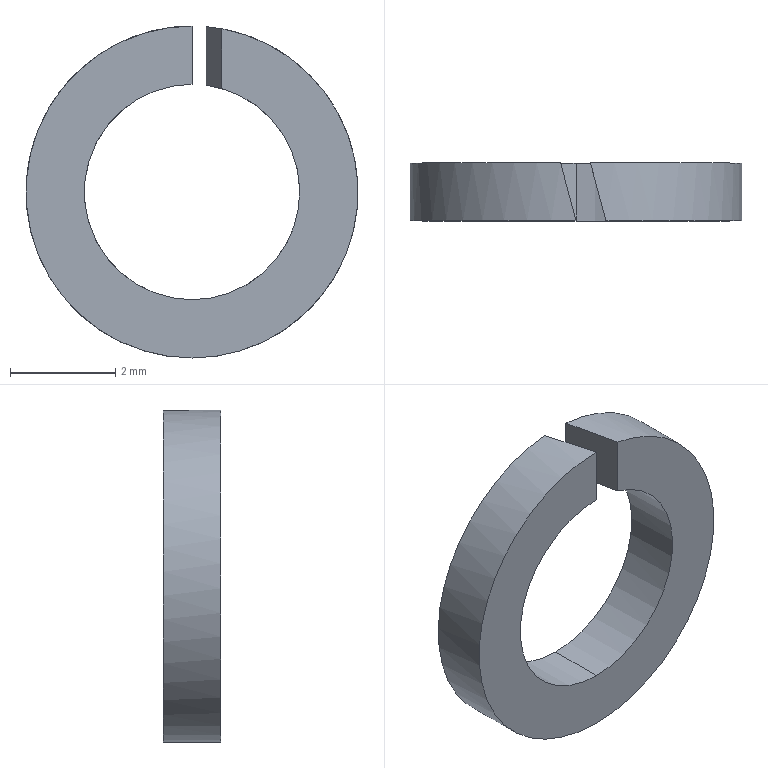Component | SolidWorks | GB 93-87-4-10 | 1 solid | 8 faces | box 6.32 x 1.1 x 6.32 mm | volume 19 mm3 | cylinder 4 | plane 4 | commonest cylinder face diameters 4.1 x2 6.32 x2
build123d program:
from build123d import *

# Parameters (mm, degrees)
SKETCH1_R               = 3.16
SKETCH1_R_2             = 2.05
BOSS_EXTRUDE1_DEPTH     = 1.1
CUT_EXTRUDE1_REACH      = 6.602
CUT_EXTRUDE1_END_RADIUS = 3.16


with BuildPart() as part:
    # Sketch1 → Boss-Extrude1 (new body)
    with BuildSketch(Plane(origin=(0, 0, 0), x_dir=(1, 0, 0), z_dir=(0, 1, 0))):
        with Locations(Location((0, 0, 0), (0, 0, 270))):
            Circle(SKETCH1_R)
        with Locations(Location((0, 0, 0), (0, 0, 270))):
            Circle(SKETCH1_R_2, mode=Mode.SUBTRACT)
    extrude(amount=BOSS_EXTRUDE1_DEPTH)

    # Cut-Extrude1: up to this cylinder (the profile starts inside it)
    cut_extrude1_end = Plane(origin=(0, 0.55, 0), z_dir=(0, -1, 0)) * Cylinder(CUT_EXTRUDE1_END_RADIUS, 20.524, mode=Mode.PRIVATE)
    # Sketch2 → Cut-Extrude1 (cut, up to the surface)
    with BuildSketch(Plane.XY, mode=Mode.PRIVATE) as cut_extrude1_sk1:
        Polygon((0, 0), (-0.2947, 1.1), (0.2747, 1.1), (0.5694, 0), align=None)
    cut_extrude1_tool1 = extrude(cut_extrude1_sk1.sketch, amount=CUT_EXTRUDE1_REACH, mode=Mode.PRIVATE) & cut_extrude1_end
    add(cut_extrude1_tool1.solids().sort_by_distance((0.1373, 0.55, 0))[0], mode=Mode.SUBTRACT)


solid = part.part

# Placed as in the assembly
solid = solid.moved(Location((-51.534, 76.366, -146.507), (0, 0, 0)))
STEP:
#1=COLOUR_RGB('',0.7922,0.8196,0.9333);
#2=FILL_AREA_STYLE_COLOUR('',#1);
#3=FILL_AREA_STYLE('',(#2));
#4=SURFACE_STYLE_FILL_AREA(#3);
#5=SURFACE_SIDE_STYLE('',(#4));
#6=SURFACE_STYLE_USAGE(.BOTH.,#5);
#7=PRESENTATION_STYLE_ASSIGNMENT((#6));
#8=CARTESIAN_POINT('',(-2.018,3.05,-5.688));
#9=VERTEX_POINT('',#8);
#10=CARTESIAN_POINT('',(-2.029,3.05,-5.849));
#11=VERTEX_POINT('',#10);
#12=CARTESIAN_POINT('',(-2.029,3.05,-5.768));
#13=DIRECTION('',(0.,1.,0.));
#14=DIRECTION('',(0.,0.,1.));
#15=AXIS2_PLACEMENT_3D('',#12,#13,#14);
#16=CIRCLE('',#15,0.08071);
#17=EDGE_CURVE('',#9,#11,#16,.T.);
#18=ORIENTED_EDGE('',*,*,#17,.T.);
#19=CARTESIAN_POINT('',(-2.029,3.007,-5.849));
#20=VERTEX_POINT('',#19);
#21=CARTESIAN_POINT('',(-2.029,3.05,-5.849));
#22=DIRECTION('',(0.,-1.,0.));
#23=VECTOR('',#22,39.37);
#24=LINE('',#21,#23);
#25=EDGE_CURVE('',#11,#20,#24,.T.);
#26=ORIENTED_EDGE('',*,*,#25,.T.);
#27=CARTESIAN_POINT('',(-2.006,3.007,-5.69));
#28=VERTEX_POINT('',#27);
#29=CARTESIAN_POINT('',(-2.029,3.007,-5.768));
#30=DIRECTION('',(0.,1.,0.));
#31=DIRECTION('',(0.,0.,1.));
#32=AXIS2_PLACEMENT_3D('',#29,#30,#31);
#33=CIRCLE('',#32,0.08071);
#34=EDGE_CURVE('',#28,#20,#33,.T.);
#35=ORIENTED_EDGE('',*,*,#34,.F.);
#36=CARTESIAN_POINT('',(-2.018,3.05,-5.688));
#37=CARTESIAN_POINT('',(-2.014,3.035,-5.689));
#38=CARTESIAN_POINT('',(-2.01,3.021,-5.689));
#39=CARTESIAN_POINT('',(-2.006,3.007,-5.69));
#40=(BOUNDED_CURVE()B_SPLINE_CURVE(3,(#36,#37,#38,#39),.UNSPECIFIED.,.F.,.F.)B_SPLINE_CURVE_WITH_KNOTS((4,4),(4.847,4.994),.UNSPECIFIED.)CURVE()GEOMETRIC_REPRESENTATION_ITEM()RATIONAL_B_SPLINE_CURVE((1.,0.9982,0.9982,1.))REPRESENTATION_ITEM(''));
#41=EDGE_CURVE('',#9,#28,#40,.T.);
#42=ORIENTED_EDGE('',*,*,#41,.F.);
#43=EDGE_LOOP('',(#18,#26,#35,#42));
#44=FACE_OUTER_BOUND('',#43,.T.);
#45=CARTESIAN_POINT('',(-2.029,3.05,-5.768));
#46=DIRECTION('',(0.,-1.,0.));
#47=DIRECTION('',(0.,0.,-1.));
#48=AXIS2_PLACEMENT_3D('',#45,#46,#47);
#49=CYLINDRICAL_SURFACE('',#48,0.08071);
#50=ADVANCED_FACE('',(#44),#49,.F.);
#51=CARTESIAN_POINT('',(-2.029,3.05,-5.892));
#52=VERTEX_POINT('',#51);
#53=CARTESIAN_POINT('',(-2.041,3.05,-5.644));
#54=VERTEX_POINT('',#53);
#55=CARTESIAN_POINT('',(-2.029,3.05,-5.768));
#56=DIRECTION('',(0.,1.,0.));
#57=DIRECTION('',(0.,0.,1.));
#58=AXIS2_PLACEMENT_3D('',#55,#56,#57);
#59=CIRCLE('',#58,0.1244);
#60=EDGE_CURVE('',#52,#54,#59,.T.);
#61=ORIENTED_EDGE('',*,*,#60,.F.);
#62=CARTESIAN_POINT('',(-2.029,3.007,-5.892));
#63=VERTEX_POINT('',#62);
#64=CARTESIAN_POINT('',(-2.029,3.05,-5.892));
#65=DIRECTION('',(0.,-1.,0.));
#66=VECTOR('',#65,39.37);
#67=LINE('',#64,#66);
#68=EDGE_CURVE('',#52,#63,#67,.T.);
#69=ORIENTED_EDGE('',*,*,#68,.T.);
#70=CARTESIAN_POINT('',(-2.029,3.007,-5.644));
#71=VERTEX_POINT('',#70);
#72=CARTESIAN_POINT('',(-2.029,3.007,-5.768));
#73=DIRECTION('',(0.,1.,0.));
#74=DIRECTION('',(0.,0.,1.));
#75=AXIS2_PLACEMENT_3D('',#72,#73,#74);
#76=CIRCLE('',#75,0.1244);
#77=EDGE_CURVE('',#63,#71,#76,.T.);
#78=ORIENTED_EDGE('',*,*,#77,.T.);
#79=CARTESIAN_POINT('',(-2.029,3.007,-5.644));
#80=CARTESIAN_POINT('',(-2.033,3.021,-5.644));
#81=CARTESIAN_POINT('',(-2.037,3.035,-5.644));
#82=CARTESIAN_POINT('',(-2.041,3.05,-5.644));
#83=(BOUNDED_CURVE()B_SPLINE_CURVE(3,(#79,#80,#81,#82),.UNSPECIFIED.,.F.,.F.)B_SPLINE_CURVE_WITH_KNOTS((4,4),(1.571,1.664),.UNSPECIFIED.)CURVE()GEOMETRIC_REPRESENTATION_ITEM()RATIONAL_B_SPLINE_CURVE((1.,0.9993,0.9993,1.))REPRESENTATION_ITEM(''));
#84=EDGE_CURVE('',#71,#54,#83,.T.);
#85=ORIENTED_EDGE('',*,*,#84,.T.);
#86=EDGE_LOOP('',(#61,#69,#78,#85));
#87=FACE_OUTER_BOUND('',#86,.T.);
#88=CARTESIAN_POINT('',(-2.029,3.05,-5.768));
#89=DIRECTION('',(0.,-1.,0.));
#90=DIRECTION('',(0.,0.,-1.));
#91=AXIS2_PLACEMENT_3D('',#88,#89,#90);
#92=CYLINDRICAL_SURFACE('',#91,0.1244);
#93=ADVANCED_FACE('',(#87),#92,.T.);
#94=ORIENTED_EDGE('',*,*,#17,.F.);
#95=CARTESIAN_POINT('',(-2.018,3.05,-5.644));
#96=VERTEX_POINT('',#95);
#97=CARTESIAN_POINT('',(-2.018,3.05,-5.644));
#98=DIRECTION('',(0.,0.,-1.));
#99=VECTOR('',#98,39.37);
#100=LINE('',#97,#99);
#101=EDGE_CURVE('',#96,#9,#100,.T.);
#102=ORIENTED_EDGE('',*,*,#101,.F.);
#103=CARTESIAN_POINT('',(-2.029,3.05,-5.768));
#104=DIRECTION('',(0.,1.,0.));
#105=DIRECTION('',(0.,0.,1.));
#106=AXIS2_PLACEMENT_3D('',#103,#104,#105);
#107=CIRCLE('',#106,0.1244);
#108=EDGE_CURVE('',#96,#52,#107,.T.);
#109=ORIENTED_EDGE('',*,*,#108,.T.);
#110=ORIENTED_EDGE('',*,*,#60,.T.);
#111=CARTESIAN_POINT('',(-2.041,3.05,-5.688));
#112=VERTEX_POINT('',#111);
#113=CARTESIAN_POINT('',(-2.041,3.05,-5.644));
#114=DIRECTION('',(0.,0.,-1.));
#115=VECTOR('',#114,39.37);
#116=LINE('',#113,#115);
#117=EDGE_CURVE('',#54,#112,#116,.T.);
#118=ORIENTED_EDGE('',*,*,#117,.T.);
#119=CARTESIAN_POINT('',(-2.029,3.05,-5.768));
#120=DIRECTION('',(0.,1.,0.));
#121=DIRECTION('',(0.,0.,1.));
#122=AXIS2_PLACEMENT_3D('',#119,#120,#121);
#123=CIRCLE('',#122,0.08071);
#124=EDGE_CURVE('',#11,#112,#123,.T.);
#125=ORIENTED_EDGE('',*,*,#124,.F.);
#126=EDGE_LOOP('',(#94,#102,#109,#110,#118,#125));
#127=FACE_OUTER_BOUND('',#126,.T.);
#128=CARTESIAN_POINT('',(-2.029,3.05,-5.768));
#129=DIRECTION('',(0.,1.,0.));
#130=DIRECTION('',(0.,0.,1.));
#131=AXIS2_PLACEMENT_3D('',#128,#129,#130);
#132=PLANE('',#131);
#133=ADVANCED_FACE('',(#127),#132,.T.);
#134=CARTESIAN_POINT('',(-2.006,3.007,-5.646));
#135=VERTEX_POINT('',#134);
#136=CARTESIAN_POINT('',(-2.006,3.007,-5.644));
#137=DIRECTION('',(0.,0.,-1.));
#138=VECTOR('',#137,39.37);
#139=LINE('',#136,#138);
#140=EDGE_CURVE('',#135,#28,#139,.T.);
#141=ORIENTED_EDGE('',*,*,#140,.T.);
#142=ORIENTED_EDGE('',*,*,#34,.T.);
#143=CARTESIAN_POINT('',(-2.029,3.007,-5.687));
#144=VERTEX_POINT('',#143);
#145=CARTESIAN_POINT('',(-2.029,3.007,-5.768));
#146=DIRECTION('',(0.,1.,0.));
#147=DIRECTION('',(0.,0.,1.));
#148=AXIS2_PLACEMENT_3D('',#145,#146,#147);
#149=CIRCLE('',#148,0.08071);
#150=EDGE_CURVE('',#20,#144,#149,.T.);
#151=ORIENTED_EDGE('',*,*,#150,.T.);
#152=CARTESIAN_POINT('',(-2.029,3.007,-5.644));
#153=DIRECTION('',(0.,0.,-1.));
#154=VECTOR('',#153,39.37);
#155=LINE('',#152,#154);
#156=EDGE_CURVE('',#71,#144,#155,.T.);
#157=ORIENTED_EDGE('',*,*,#156,.F.);
#158=ORIENTED_EDGE('',*,*,#77,.F.);
#159=CARTESIAN_POINT('',(-2.029,3.007,-5.768));
#160=DIRECTION('',(0.,1.,0.));
#161=DIRECTION('',(0.,0.,1.));
#162=AXIS2_PLACEMENT_3D('',#159,#160,#161);
#163=CIRCLE('',#162,0.1244);
#164=EDGE_CURVE('',#135,#63,#163,.T.);
#165=ORIENTED_EDGE('',*,*,#164,.F.);
#166=EDGE_LOOP('',(#141,#142,#151,#157,#158,#165));
#167=FACE_OUTER_BOUND('',#166,.T.);
#168=CARTESIAN_POINT('',(-2.029,3.007,-5.768));
#169=DIRECTION('',(0.,1.,0.));
#170=DIRECTION('',(0.,0.,1.));
#171=AXIS2_PLACEMENT_3D('',#168,#169,#170);
#172=PLANE('',#171);
#173=ADVANCED_FACE('',(#167),#172,.F.);
#174=ORIENTED_EDGE('',*,*,#68,.F.);
#175=ORIENTED_EDGE('',*,*,#108,.F.);
#176=CARTESIAN_POINT('',(-2.018,3.05,-5.644));
#177=CARTESIAN_POINT('',(-2.014,3.035,-5.644));
#178=CARTESIAN_POINT('',(-2.01,3.021,-5.645));
#179=CARTESIAN_POINT('',(-2.006,3.007,-5.646));
#180=(BOUNDED_CURVE()B_SPLINE_CURVE(3,(#176,#177,#178,#179),.UNSPECIFIED.,.F.,.F.)B_SPLINE_CURVE_WITH_KNOTS((4,4),(4.799,4.894),.UNSPECIFIED.)CURVE()GEOMETRIC_REPRESENTATION_ITEM()RATIONAL_B_SPLINE_CURVE((1.,0.9993,0.9993,1.))REPRESENTATION_ITEM(''));
#181=EDGE_CURVE('',#96,#135,#180,.T.);
#182=ORIENTED_EDGE('',*,*,#181,.T.);
#183=ORIENTED_EDGE('',*,*,#164,.T.);
#184=EDGE_LOOP('',(#174,#175,#182,#183));
#185=FACE_OUTER_BOUND('',#184,.T.);
#186=CARTESIAN_POINT('',(-2.029,3.05,-5.768));
#187=DIRECTION('',(0.,-1.,0.));
#188=DIRECTION('',(0.,0.,-1.));
#189=AXIS2_PLACEMENT_3D('',#186,#187,#188);
#190=CYLINDRICAL_SURFACE('',#189,0.1244);
#191=ADVANCED_FACE('',(#185),#190,.T.);
#192=ORIENTED_EDGE('',*,*,#25,.F.);
#193=ORIENTED_EDGE('',*,*,#124,.T.);
#194=CARTESIAN_POINT('',(-2.029,3.007,-5.687));
#195=CARTESIAN_POINT('',(-2.033,3.021,-5.687));
#196=CARTESIAN_POINT('',(-2.037,3.035,-5.688));
#197=CARTESIAN_POINT('',(-2.041,3.05,-5.688));
#198=(BOUNDED_CURVE()B_SPLINE_CURVE(3,(#194,#195,#196,#197),.UNSPECIFIED.,.F.,.F.)B_SPLINE_CURVE_WITH_KNOTS((4,4),(1.571,1.715),.UNSPECIFIED.)CURVE()GEOMETRIC_REPRESENTATION_ITEM()RATIONAL_B_SPLINE_CURVE((1.,0.9983,0.9983,1.))REPRESENTATION_ITEM(''));
#199=EDGE_CURVE('',#144,#112,#198,.T.);
#200=ORIENTED_EDGE('',*,*,#199,.F.);
#201=ORIENTED_EDGE('',*,*,#150,.F.);
#202=EDGE_LOOP('',(#192,#193,#200,#201));
#203=FACE_OUTER_BOUND('',#202,.T.);
#204=CARTESIAN_POINT('',(-2.029,3.05,-5.768));
#205=DIRECTION('',(0.,-1.,0.));
#206=DIRECTION('',(0.,0.,-1.));
#207=AXIS2_PLACEMENT_3D('',#204,#205,#206);
#208=CYLINDRICAL_SURFACE('',#207,0.08071);
#209=ADVANCED_FACE('',(#203),#208,.F.);
#210=ORIENTED_EDGE('',*,*,#156,.T.);
#211=ORIENTED_EDGE('',*,*,#199,.T.);
#212=ORIENTED_EDGE('',*,*,#117,.F.);
#213=ORIENTED_EDGE('',*,*,#84,.F.);
#214=EDGE_LOOP('',(#210,#211,#212,#213));
#215=FACE_OUTER_BOUND('',#214,.T.);
#216=CARTESIAN_POINT('',(-2.029,3.007,-5.644));
#217=DIRECTION('',(0.9659,0.2588,0.));
#218=DIRECTION('',(-0.2588,0.9659,0.));
#219=AXIS2_PLACEMENT_3D('',#216,#217,#218);
#220=PLANE('',#219);
#221=ADVANCED_FACE('',(#215),#220,.T.);
#222=ORIENTED_EDGE('',*,*,#101,.T.);
#223=ORIENTED_EDGE('',*,*,#41,.T.);
#224=ORIENTED_EDGE('',*,*,#140,.F.);
#225=ORIENTED_EDGE('',*,*,#181,.F.);
#226=EDGE_LOOP('',(#222,#223,#224,#225));
#227=FACE_OUTER_BOUND('',#226,.T.);
#228=CARTESIAN_POINT('',(-2.006,3.007,-5.644));
#229=DIRECTION('',(-0.9659,-0.2588,0.));
#230=DIRECTION('',(0.2588,-0.9659,0.));
#231=AXIS2_PLACEMENT_3D('',#228,#229,#230);
#232=PLANE('',#231);
#233=ADVANCED_FACE('',(#227),#232,.T.);
#234=CLOSED_SHELL('',(#50,#93,#133,#173,#191,#209,#221,#233));
#235=MANIFOLD_SOLID_BREP('',#234);
#236=STYLED_ITEM('',(#7),#235);
#237=PRESENTATION_LAYER_ASSIGNMENT('','',(#236));
#238=(LENGTH_UNIT()NAMED_UNIT(*)SI_UNIT($,.METRE.));
#239=LENGTH_MEASURE_WITH_UNIT(LENGTH_MEASURE(0.0254),#238);
#240=DIMENSIONAL_EXPONENTS(1.,0.,0.,0.,0.,0.,0.);
#241=(CONVERSION_BASED_UNIT('',#239)LENGTH_UNIT()NAMED_UNIT(#240));
#242=UNCERTAINTY_MEASURE_WITH_UNIT(LENGTH_MEASURE(0.00001),#241,'','');
#243=(NAMED_UNIT(*)PLANE_ANGLE_UNIT()SI_UNIT($,.RADIAN.));
#244=(NAMED_UNIT(*)SI_UNIT($,.STERADIAN.)SOLID_ANGLE_UNIT());
#245=(GEOMETRIC_REPRESENTATION_CONTEXT(3)GLOBAL_UNCERTAINTY_ASSIGNED_CONTEXT((#242))GLOBAL_UNIT_ASSIGNED_CONTEXT((#241,#243,#244))REPRESENTATION_CONTEXT('',''));
#246=MECHANICAL_DESIGN_GEOMETRIC_PRESENTATION_REPRESENTATION('',(#236),#245);
#247=CARTESIAN_POINT('',(0.,0.,0.));
#248=DIRECTION('',(0.,0.,1.));
#249=DIRECTION('',(1.,0.,0.));
#250=AXIS2_PLACEMENT_3D('',#247,#248,#249);
#251=(LENGTH_UNIT()NAMED_UNIT(*)SI_UNIT($,.METRE.));
#252=LENGTH_MEASURE_WITH_UNIT(LENGTH_MEASURE(0.0254),#251);
#253=DIMENSIONAL_EXPONENTS(1.,0.,0.,0.,0.,0.,0.);
#254=(CONVERSION_BASED_UNIT('',#252)LENGTH_UNIT()NAMED_UNIT(#253));
#255=UNCERTAINTY_MEASURE_WITH_UNIT(LENGTH_MEASURE(0.00001),#254,'','');
#256=(NAMED_UNIT(*)PLANE_ANGLE_UNIT()SI_UNIT($,.RADIAN.));
#257=(NAMED_UNIT(*)SI_UNIT($,.STERADIAN.)SOLID_ANGLE_UNIT());
#258=(GEOMETRIC_REPRESENTATION_CONTEXT(3)GLOBAL_UNCERTAINTY_ASSIGNED_CONTEXT((#255))GLOBAL_UNIT_ASSIGNED_CONTEXT((#254,#256,#257))REPRESENTATION_CONTEXT('',''));
#259=ADVANCED_BREP_SHAPE_REPRESENTATION('',(#235,#250),#258);